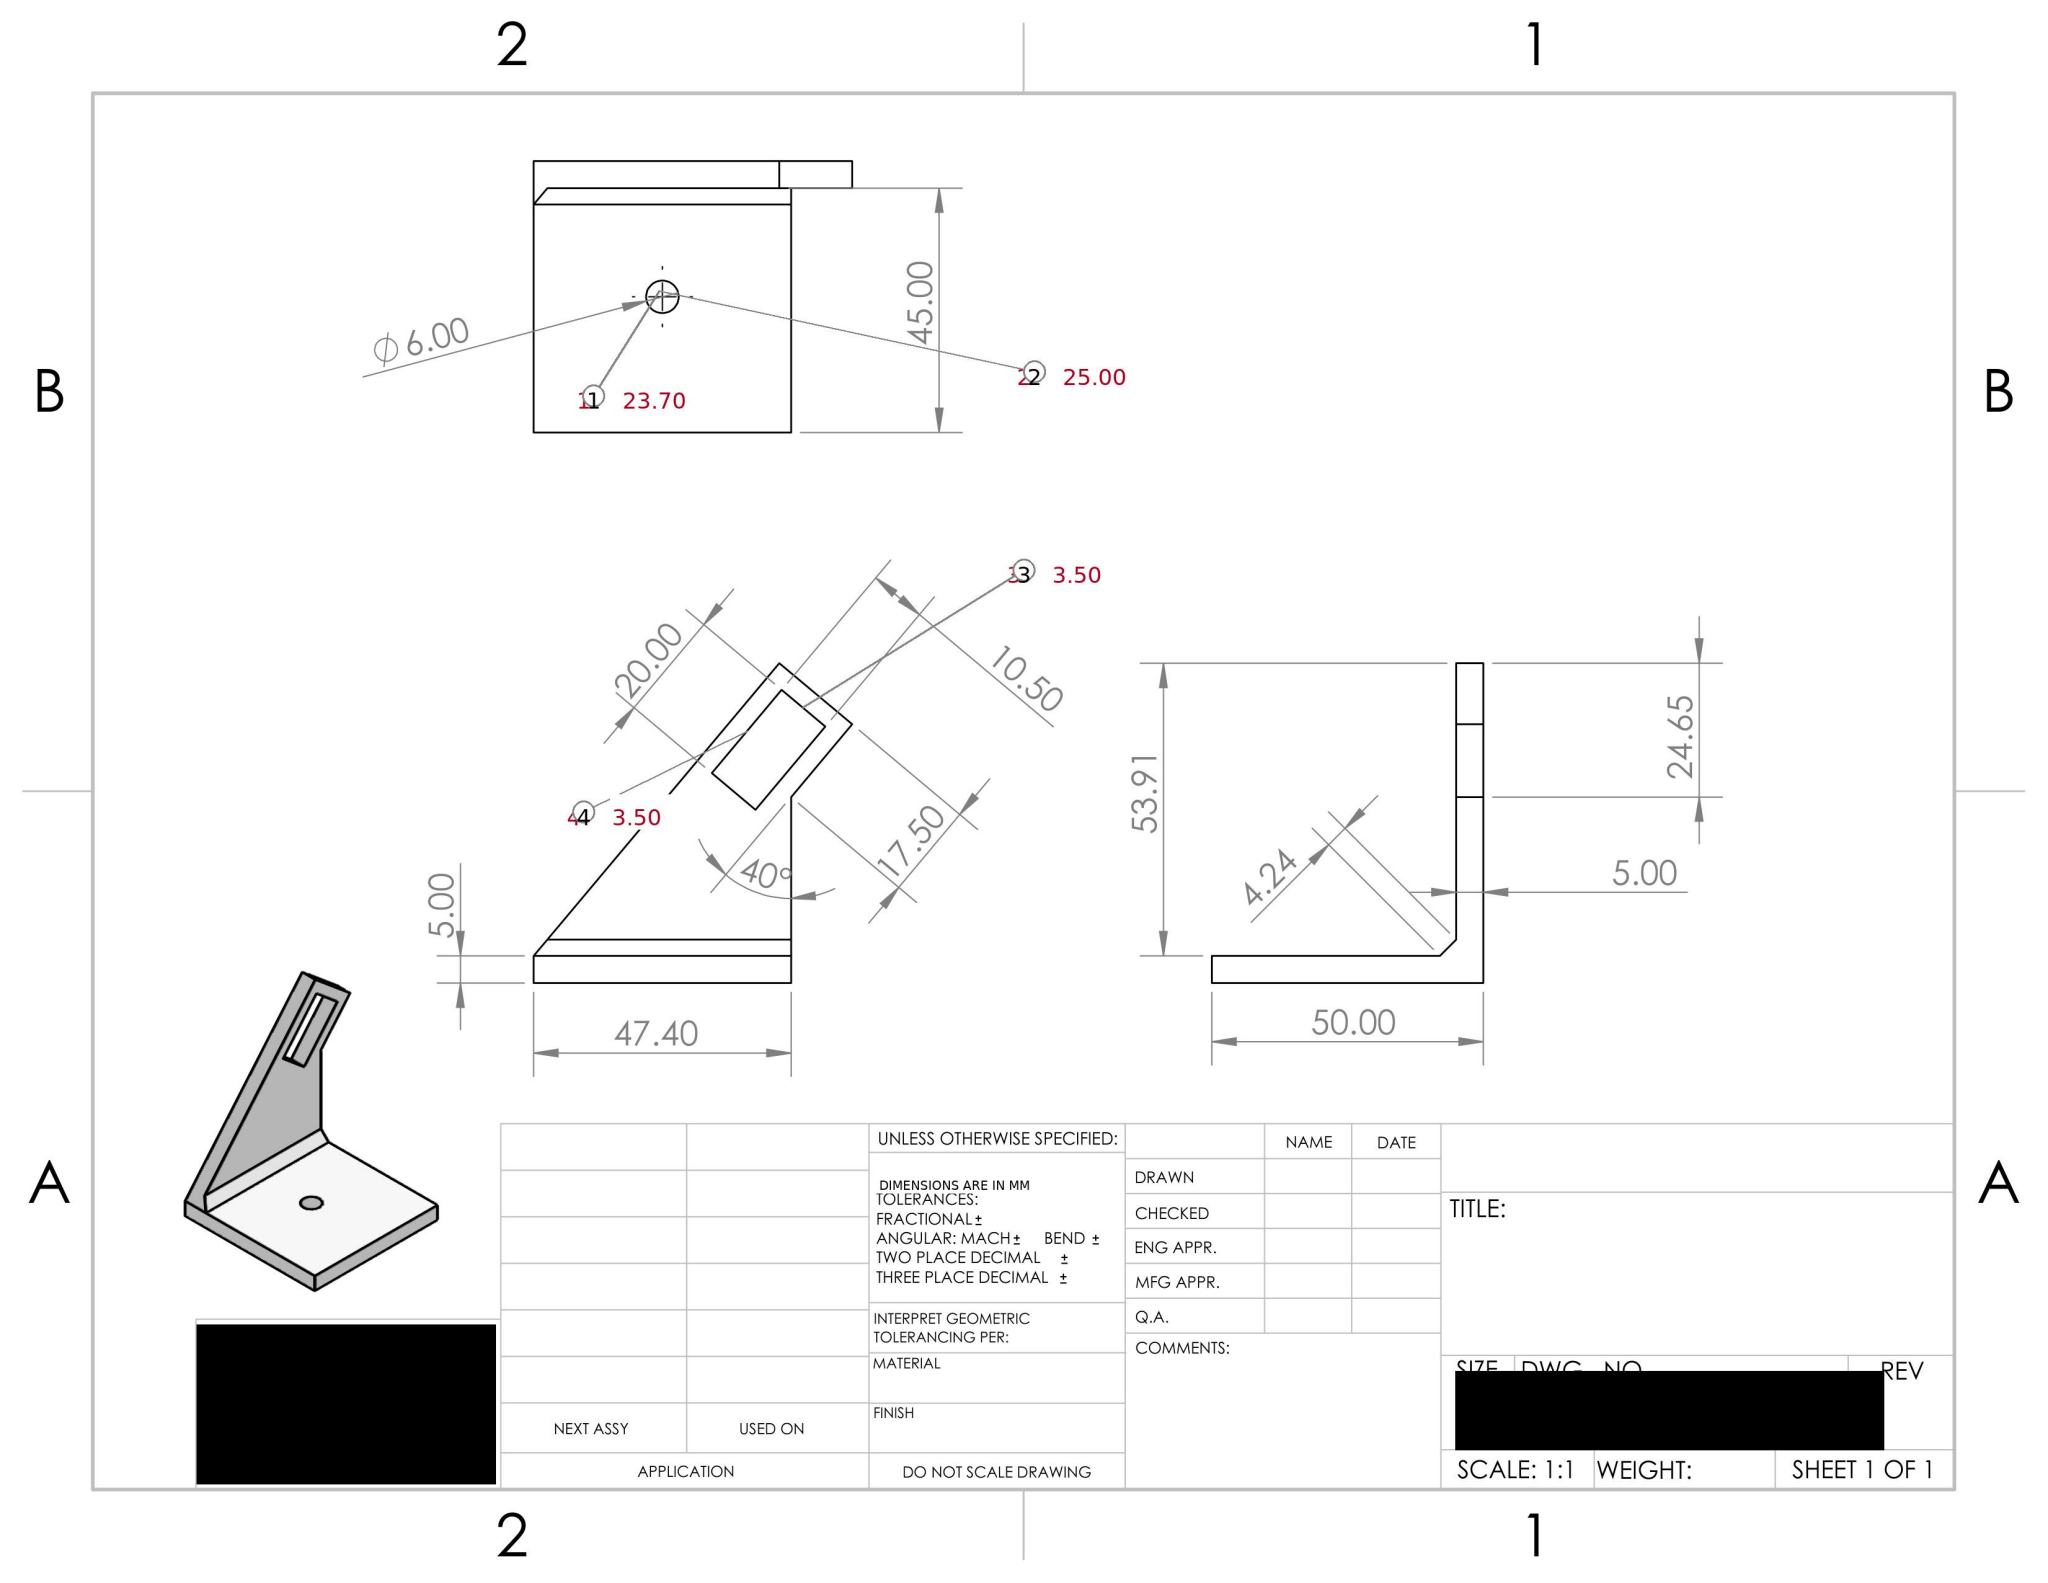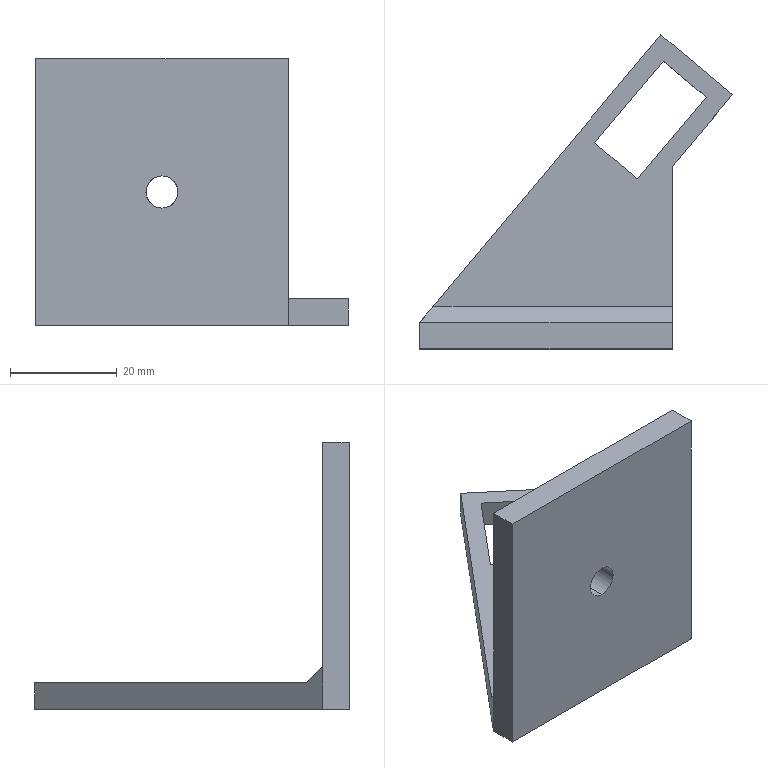Part | SolidWorks | mm | 1 solid | 17 faces | box 58.65 x 58.91 x 50 mm | volume 18179 mm3 | plane 15 | cylinder 2 | commonest cylinder face diameters 6 x2
STEP:
#1=CARTESIAN_POINT('',(23.698,0.,19.5));
#2=VERTEX_POINT('',#1);
#3=CARTESIAN_POINT('',(23.698,0.,25.5));
#4=VERTEX_POINT('',#3);
#5=CARTESIAN_POINT('',(23.698,0.,22.5));
#6=DIRECTION('',(0.,1.,0.));
#7=DIRECTION('',(0.,0.,1.));
#8=AXIS2_PLACEMENT_3D('',#5,#6,#7);
#9=CIRCLE('',#8,3.);
#10=EDGE_CURVE('',#2,#4,#9,.T.);
#11=ORIENTED_EDGE('',*,*,#10,.T.);
#12=CARTESIAN_POINT('',(23.698,-5.,25.5));
#13=VERTEX_POINT('',#12);
#14=CARTESIAN_POINT('',(23.698,53.914,25.5));
#15=DIRECTION('',(0.,-1.,0.));
#16=VECTOR('',#15,1000.);
#17=LINE('',#14,#16);
#18=EDGE_CURVE('',#4,#13,#17,.T.);
#19=ORIENTED_EDGE('',*,*,#18,.T.);
#20=CARTESIAN_POINT('',(23.698,-5.,19.5));
#21=VERTEX_POINT('',#20);
#22=CARTESIAN_POINT('',(23.698,-5.,25.5));
#23=CARTESIAN_POINT('',(23.305,-5.,25.5));
#24=CARTESIAN_POINT('',(22.913,-5.,25.422));
#25=CARTESIAN_POINT('',(22.187,-5.,25.121));
#26=CARTESIAN_POINT('',(21.854,-5.,24.899));
#27=CARTESIAN_POINT('',(21.299,-5.,24.344));
#28=CARTESIAN_POINT('',(21.077,-5.,24.011));
#29=CARTESIAN_POINT('',(20.776,-5.,23.285));
#30=CARTESIAN_POINT('',(20.698,-5.,22.893));
#31=CARTESIAN_POINT('',(20.698,-5.,22.107));
#32=CARTESIAN_POINT('',(20.776,-5.,21.715));
#33=CARTESIAN_POINT('',(21.077,-5.,20.989));
#34=CARTESIAN_POINT('',(21.299,-5.,20.656));
#35=CARTESIAN_POINT('',(21.854,-5.,20.101));
#36=CARTESIAN_POINT('',(22.187,-5.,19.879));
#37=CARTESIAN_POINT('',(22.913,-5.,19.578));
#38=CARTESIAN_POINT('',(23.305,-5.,19.5));
#39=CARTESIAN_POINT('',(23.698,-5.,19.5));
#40=B_SPLINE_CURVE_WITH_KNOTS('',3,(#22,#23,#24,#25,#26,#27,#28,#29,#30,#31,#32,#33,#34,#35,#36,#37,#38,#39),.UNSPECIFIED.,.F.,.F.,(4,2,2,2,2,2,2,2,4),(0.5,0.5625,0.625,0.6875,0.75,0.8125,0.875,0.9375,1.),.UNSPECIFIED.);
#41=EDGE_CURVE('',#13,#21,#40,.T.);
#42=ORIENTED_EDGE('',*,*,#41,.T.);
#43=CARTESIAN_POINT('',(23.698,53.914,19.5));
#44=DIRECTION('',(0.,-1.,0.));
#45=VECTOR('',#44,1000.);
#46=LINE('',#43,#45);
#47=EDGE_CURVE('',#2,#21,#46,.T.);
#48=ORIENTED_EDGE('',*,*,#47,.F.);
#49=EDGE_LOOP('',(#11,#19,#42,#48));
#50=FACE_OUTER_BOUND('',#49,.T.);
#51=CARTESIAN_POINT('',(23.698,53.914,22.5));
#52=DIRECTION('',(0.,-1.,0.));
#53=DIRECTION('',(0.,0.,-1.));
#54=AXIS2_PLACEMENT_3D('',#51,#52,#53);
#55=CYLINDRICAL_SURFACE('',#54,3.);
#56=ADVANCED_FACE('',(#50),#55,.F.);
#57=CARTESIAN_POINT('',(0.,-5.,47.5));
#58=VERTEX_POINT('',#57);
#59=CARTESIAN_POINT('',(0.,-5.,-2.5));
#60=VERTEX_POINT('',#59);
#61=CARTESIAN_POINT('',(0.,-5.,-2.5));
#62=DIRECTION('',(0.,0.,-1.));
#63=VECTOR('',#62,1000.);
#64=LINE('',#61,#63);
#65=EDGE_CURVE('',#58,#60,#64,.T.);
#66=ORIENTED_EDGE('',*,*,#65,.T.);
#67=CARTESIAN_POINT('',(47.396,-5.,-2.5));
#68=VERTEX_POINT('',#67);
#69=CARTESIAN_POINT('',(0.,-5.,-2.5));
#70=DIRECTION('',(1.,0.,0.));
#71=VECTOR('',#70,1000.);
#72=LINE('',#69,#71);
#73=EDGE_CURVE('',#60,#68,#72,.T.);
#74=ORIENTED_EDGE('',*,*,#73,.T.);
#75=CARTESIAN_POINT('',(47.396,-5.,47.5));
#76=VERTEX_POINT('',#75);
#77=CARTESIAN_POINT('',(47.396,-5.,-2.5));
#78=DIRECTION('',(0.,0.,1.));
#79=VECTOR('',#78,1000.);
#80=LINE('',#77,#79);
#81=EDGE_CURVE('',#68,#76,#80,.T.);
#82=ORIENTED_EDGE('',*,*,#81,.T.);
#83=CARTESIAN_POINT('',(0.,-5.,47.5));
#84=DIRECTION('',(-1.,0.,0.));
#85=VECTOR('',#84,1000.);
#86=LINE('',#83,#85);
#87=EDGE_CURVE('',#76,#58,#86,.T.);
#88=ORIENTED_EDGE('',*,*,#87,.T.);
#89=EDGE_LOOP('',(#66,#74,#82,#88));
#90=FACE_OUTER_BOUND('',#89,.T.);
#91=CARTESIAN_POINT('',(23.698,-5.,19.5));
#92=CARTESIAN_POINT('',(24.091,-5.,19.5));
#93=CARTESIAN_POINT('',(24.483,-5.,19.578));
#94=CARTESIAN_POINT('',(25.209,-5.,19.879));
#95=CARTESIAN_POINT('',(25.542,-5.,20.101));
#96=CARTESIAN_POINT('',(26.097,-5.,20.656));
#97=CARTESIAN_POINT('',(26.319,-5.,20.989));
#98=CARTESIAN_POINT('',(26.62,-5.,21.715));
#99=CARTESIAN_POINT('',(26.698,-5.,22.107));
#100=CARTESIAN_POINT('',(26.698,-5.,22.893));
#101=CARTESIAN_POINT('',(26.62,-5.,23.285));
#102=CARTESIAN_POINT('',(26.319,-5.,24.011));
#103=CARTESIAN_POINT('',(26.097,-5.,24.344));
#104=CARTESIAN_POINT('',(25.542,-5.,24.899));
#105=CARTESIAN_POINT('',(25.209,-5.,25.121));
#106=CARTESIAN_POINT('',(24.483,-5.,25.422));
#107=CARTESIAN_POINT('',(24.091,-5.,25.5));
#108=CARTESIAN_POINT('',(23.698,-5.,25.5));
#109=B_SPLINE_CURVE_WITH_KNOTS('',3,(#91,#92,#93,#94,#95,#96,#97,#98,#99,#100,#101,#102,#103,#104,#105,#106,#107,#108),.UNSPECIFIED.,.F.,.F.,(4,2,2,2,2,2,2,2,4),(0.,0.0625,0.125,0.1875,0.25,0.3125,0.375,0.4375,0.5),.UNSPECIFIED.);
#110=EDGE_CURVE('',#21,#13,#109,.T.);
#111=ORIENTED_EDGE('',*,*,#110,.F.);
#112=ORIENTED_EDGE('',*,*,#41,.F.);
#113=EDGE_LOOP('',(#111,#112));
#114=FACE_BOUND('',#113,.T.);
#115=CARTESIAN_POINT('',(0.,-5.,0.));
#116=DIRECTION('',(0.,1.,0.));
#117=DIRECTION('',(0.,0.,1.));
#118=AXIS2_PLACEMENT_3D('',#115,#116,#117);
#119=PLANE('',#118);
#120=ADVANCED_FACE('',(#90,#114),#119,.F.);
#121=CARTESIAN_POINT('',(45.239,53.914,2.5));
#122=VERTEX_POINT('',#121);
#123=CARTESIAN_POINT('',(2.517,3.,2.5));
#124=VERTEX_POINT('',#123);
#125=CARTESIAN_POINT('',(0.,0.,2.5));
#126=DIRECTION('',(-0.6428,-0.766,0.));
#127=VECTOR('',#126,1000.);
#128=LINE('',#125,#127);
#129=EDGE_CURVE('',#122,#124,#128,.T.);
#130=ORIENTED_EDGE('',*,*,#129,.T.);
#131=CARTESIAN_POINT('',(47.396,3.,2.5));
#132=VERTEX_POINT('',#131);
#133=CARTESIAN_POINT('',(0.,3.,2.5));
#134=DIRECTION('',(1.,0.,0.));
#135=VECTOR('',#134,1000.);
#136=LINE('',#133,#135);
#137=EDGE_CURVE('',#124,#132,#136,.T.);
#138=ORIENTED_EDGE('',*,*,#137,.T.);
#139=CARTESIAN_POINT('',(47.396,29.259,2.5));
#140=VERTEX_POINT('',#139);
#141=CARTESIAN_POINT('',(47.396,29.259,2.5));
#142=DIRECTION('',(0.,1.,0.));
#143=VECTOR('',#142,1000.);
#144=LINE('',#141,#143);
#145=EDGE_CURVE('',#132,#140,#144,.T.);
#146=ORIENTED_EDGE('',*,*,#145,.T.);
#147=CARTESIAN_POINT('',(58.645,42.665,2.5));
#148=VERTEX_POINT('',#147);
#149=CARTESIAN_POINT('',(58.645,42.665,2.5));
#150=DIRECTION('',(0.6428,0.766,0.));
#151=VECTOR('',#150,1000.);
#152=LINE('',#149,#151);
#153=EDGE_CURVE('',#140,#148,#152,.T.);
#154=ORIENTED_EDGE('',*,*,#153,.T.);
#155=CARTESIAN_POINT('',(45.239,53.914,2.5));
#156=DIRECTION('',(-0.766,0.6428,0.));
#157=VECTOR('',#156,1000.);
#158=LINE('',#155,#157);
#159=EDGE_CURVE('',#148,#122,#158,.T.);
#160=ORIENTED_EDGE('',*,*,#159,.T.);
#161=EDGE_LOOP('',(#130,#138,#146,#154,#160));
#162=FACE_OUTER_BOUND('',#161,.T.);
#163=CARTESIAN_POINT('',(53.714,42.234,2.5));
#164=VERTEX_POINT('',#163);
#165=CARTESIAN_POINT('',(45.671,48.983,2.5));
#166=VERTEX_POINT('',#165);
#167=CARTESIAN_POINT('',(45.671,48.983,2.5));
#168=DIRECTION('',(-0.766,0.6428,0.));
#169=VECTOR('',#168,1000.);
#170=LINE('',#167,#169);
#171=EDGE_CURVE('',#164,#166,#170,.T.);
#172=ORIENTED_EDGE('',*,*,#171,.F.);
#173=CARTESIAN_POINT('',(40.858,26.913,2.5));
#174=VERTEX_POINT('',#173);
#175=CARTESIAN_POINT('',(53.714,42.234,2.5));
#176=DIRECTION('',(0.6428,0.766,0.));
#177=VECTOR('',#176,1000.);
#178=LINE('',#175,#177);
#179=EDGE_CURVE('',#174,#164,#178,.T.);
#180=ORIENTED_EDGE('',*,*,#179,.F.);
#181=CARTESIAN_POINT('',(32.815,33.662,2.5));
#182=VERTEX_POINT('',#181);
#183=CARTESIAN_POINT('',(32.815,33.662,2.5));
#184=DIRECTION('',(0.766,-0.6428,0.));
#185=VECTOR('',#184,1000.);
#186=LINE('',#183,#185);
#187=EDGE_CURVE('',#182,#174,#186,.T.);
#188=ORIENTED_EDGE('',*,*,#187,.F.);
#189=CARTESIAN_POINT('',(45.671,48.983,2.5));
#190=DIRECTION('',(-0.6428,-0.766,0.));
#191=VECTOR('',#190,1000.);
#192=LINE('',#189,#191);
#193=EDGE_CURVE('',#166,#182,#192,.T.);
#194=ORIENTED_EDGE('',*,*,#193,.F.);
#195=EDGE_LOOP('',(#172,#180,#188,#194));
#196=FACE_BOUND('',#195,.T.);
#197=CARTESIAN_POINT('',(0.,0.,2.5));
#198=DIRECTION('',(0.,0.,-1.));
#199=DIRECTION('',(-1.,0.,0.));
#200=AXIS2_PLACEMENT_3D('',#197,#198,#199);
#201=PLANE('',#200);
#202=ADVANCED_FACE('',(#162,#196),#201,.F.);
#203=CARTESIAN_POINT('',(47.396,29.259,-2.5));
#204=VERTEX_POINT('',#203);
#205=CARTESIAN_POINT('',(47.396,29.259,-2.5));
#206=DIRECTION('',(0.,1.,0.));
#207=VECTOR('',#206,1000.);
#208=LINE('',#205,#207);
#209=EDGE_CURVE('',#68,#204,#208,.T.);
#210=ORIENTED_EDGE('',*,*,#209,.F.);
#211=ORIENTED_EDGE('',*,*,#73,.F.);
#212=CARTESIAN_POINT('',(0.,0.,-2.5));
#213=VERTEX_POINT('',#212);
#214=CARTESIAN_POINT('',(0.,-5.,-2.5));
#215=DIRECTION('',(0.,1.,0.));
#216=VECTOR('',#215,1000.);
#217=LINE('',#214,#216);
#218=EDGE_CURVE('',#60,#213,#217,.T.);
#219=ORIENTED_EDGE('',*,*,#218,.T.);
#220=CARTESIAN_POINT('',(45.239,53.914,-2.5));
#221=VERTEX_POINT('',#220);
#222=CARTESIAN_POINT('',(0.,0.,-2.5));
#223=DIRECTION('',(-0.6428,-0.766,0.));
#224=VECTOR('',#223,1000.);
#225=LINE('',#222,#224);
#226=EDGE_CURVE('',#221,#213,#225,.T.);
#227=ORIENTED_EDGE('',*,*,#226,.F.);
#228=CARTESIAN_POINT('',(58.645,42.665,-2.5));
#229=VERTEX_POINT('',#228);
#230=CARTESIAN_POINT('',(45.239,53.914,-2.5));
#231=DIRECTION('',(-0.766,0.6428,0.));
#232=VECTOR('',#231,1000.);
#233=LINE('',#230,#232);
#234=EDGE_CURVE('',#229,#221,#233,.T.);
#235=ORIENTED_EDGE('',*,*,#234,.F.);
#236=CARTESIAN_POINT('',(58.645,42.665,-2.5));
#237=DIRECTION('',(0.6428,0.766,0.));
#238=VECTOR('',#237,1000.);
#239=LINE('',#236,#238);
#240=EDGE_CURVE('',#204,#229,#239,.T.);
#241=ORIENTED_EDGE('',*,*,#240,.F.);
#242=EDGE_LOOP('',(#210,#211,#219,#227,#235,#241));
#243=FACE_OUTER_BOUND('',#242,.T.);
#244=CARTESIAN_POINT('',(40.858,26.913,-2.5));
#245=VERTEX_POINT('',#244);
#246=CARTESIAN_POINT('',(53.714,42.234,-2.5));
#247=VERTEX_POINT('',#246);
#248=CARTESIAN_POINT('',(53.714,42.234,-2.5));
#249=DIRECTION('',(0.6428,0.766,0.));
#250=VECTOR('',#249,1000.);
#251=LINE('',#248,#250);
#252=EDGE_CURVE('',#245,#247,#251,.T.);
#253=ORIENTED_EDGE('',*,*,#252,.T.);
#254=CARTESIAN_POINT('',(45.671,48.983,-2.5));
#255=VERTEX_POINT('',#254);
#256=CARTESIAN_POINT('',(45.671,48.983,-2.5));
#257=DIRECTION('',(-0.766,0.6428,0.));
#258=VECTOR('',#257,1000.);
#259=LINE('',#256,#258);
#260=EDGE_CURVE('',#247,#255,#259,.T.);
#261=ORIENTED_EDGE('',*,*,#260,.T.);
#262=CARTESIAN_POINT('',(32.815,33.662,-2.5));
#263=VERTEX_POINT('',#262);
#264=CARTESIAN_POINT('',(45.671,48.983,-2.5));
#265=DIRECTION('',(-0.6428,-0.766,0.));
#266=VECTOR('',#265,1000.);
#267=LINE('',#264,#266);
#268=EDGE_CURVE('',#255,#263,#267,.T.);
#269=ORIENTED_EDGE('',*,*,#268,.T.);
#270=CARTESIAN_POINT('',(32.815,33.662,-2.5));
#271=DIRECTION('',(0.766,-0.6428,0.));
#272=VECTOR('',#271,1000.);
#273=LINE('',#270,#272);
#274=EDGE_CURVE('',#263,#245,#273,.T.);
#275=ORIENTED_EDGE('',*,*,#274,.T.);
#276=EDGE_LOOP('',(#253,#261,#269,#275));
#277=FACE_BOUND('',#276,.T.);
#278=CARTESIAN_POINT('',(0.,0.,-2.5));
#279=DIRECTION('',(0.,0.,-1.));
#280=DIRECTION('',(-1.,0.,0.));
#281=AXIS2_PLACEMENT_3D('',#278,#279,#280);
#282=PLANE('',#281);
#283=ADVANCED_FACE('',(#243,#277),#282,.T.);
#284=ORIENTED_EDGE('',*,*,#209,.T.);
#285=CARTESIAN_POINT('',(47.396,29.259,2.5));
#286=DIRECTION('',(0.,0.,-1.));
#287=VECTOR('',#286,1000.);
#288=LINE('',#285,#287);
#289=EDGE_CURVE('',#140,#204,#288,.T.);
#290=ORIENTED_EDGE('',*,*,#289,.F.);
#291=ORIENTED_EDGE('',*,*,#145,.F.);
#292=CARTESIAN_POINT('',(47.396,0.,5.5));
#293=VERTEX_POINT('',#292);
#294=CARTESIAN_POINT('',(47.396,16.13,-10.63));
#295=DIRECTION('',(0.,-0.7071,0.7071));
#296=VECTOR('',#295,1000.);
#297=LINE('',#294,#296);
#298=EDGE_CURVE('',#132,#293,#297,.T.);
#299=ORIENTED_EDGE('',*,*,#298,.T.);
#300=CARTESIAN_POINT('',(47.396,0.,47.5));
#301=VERTEX_POINT('',#300);
#302=CARTESIAN_POINT('',(47.396,0.,-2.5));
#303=DIRECTION('',(0.,0.,1.));
#304=VECTOR('',#303,1000.);
#305=LINE('',#302,#304);
#306=EDGE_CURVE('',#293,#301,#305,.T.);
#307=ORIENTED_EDGE('',*,*,#306,.T.);
#308=CARTESIAN_POINT('',(47.396,-5.,47.5));
#309=DIRECTION('',(0.,1.,0.));
#310=VECTOR('',#309,1000.);
#311=LINE('',#308,#310);
#312=EDGE_CURVE('',#76,#301,#311,.T.);
#313=ORIENTED_EDGE('',*,*,#312,.F.);
#314=ORIENTED_EDGE('',*,*,#81,.F.);
#315=EDGE_LOOP('',(#284,#290,#291,#299,#307,#313,#314));
#316=FACE_OUTER_BOUND('',#315,.T.);
#317=CARTESIAN_POINT('',(47.396,29.259,2.5));
#318=DIRECTION('',(-1.,0.,0.));
#319=DIRECTION('',(0.,0.,1.));
#320=AXIS2_PLACEMENT_3D('',#317,#318,#319);
#321=PLANE('',#320);
#322=ADVANCED_FACE('',(#316),#321,.F.);
#323=ORIENTED_EDGE('',*,*,#240,.T.);
#324=CARTESIAN_POINT('',(58.645,42.665,2.5));
#325=DIRECTION('',(0.,0.,-1.));
#326=VECTOR('',#325,1000.);
#327=LINE('',#324,#326);
#328=EDGE_CURVE('',#148,#229,#327,.T.);
#329=ORIENTED_EDGE('',*,*,#328,.F.);
#330=ORIENTED_EDGE('',*,*,#153,.F.);
#331=ORIENTED_EDGE('',*,*,#289,.T.);
#332=EDGE_LOOP('',(#323,#329,#330,#331));
#333=FACE_OUTER_BOUND('',#332,.T.);
#334=CARTESIAN_POINT('',(58.645,42.665,2.5));
#335=DIRECTION('',(-0.766,0.6428,0.));
#336=DIRECTION('',(-0.6428,-0.766,0.));
#337=AXIS2_PLACEMENT_3D('',#334,#335,#336);
#338=PLANE('',#337);
#339=ADVANCED_FACE('',(#333),#338,.F.);
#340=ORIENTED_EDGE('',*,*,#234,.T.);
#341=CARTESIAN_POINT('',(45.239,53.914,2.5));
#342=DIRECTION('',(0.,0.,-1.));
#343=VECTOR('',#342,1000.);
#344=LINE('',#341,#343);
#345=EDGE_CURVE('',#122,#221,#344,.T.);
#346=ORIENTED_EDGE('',*,*,#345,.F.);
#347=ORIENTED_EDGE('',*,*,#159,.F.);
#348=ORIENTED_EDGE('',*,*,#328,.T.);
#349=EDGE_LOOP('',(#340,#346,#347,#348));
#350=FACE_OUTER_BOUND('',#349,.T.);
#351=CARTESIAN_POINT('',(45.239,53.914,2.5));
#352=DIRECTION('',(-0.6428,-0.766,0.));
#353=DIRECTION('',(0.766,-0.6428,0.));
#354=AXIS2_PLACEMENT_3D('',#351,#352,#353);
#355=PLANE('',#354);
#356=ADVANCED_FACE('',(#350),#355,.F.);
#357=ORIENTED_EDGE('',*,*,#226,.T.);
#358=CARTESIAN_POINT('',(0.,0.,5.5));
#359=VERTEX_POINT('',#358);
#360=CARTESIAN_POINT('',(0.,0.,2.5));
#361=DIRECTION('',(0.,0.,-1.));
#362=VECTOR('',#361,1000.);
#363=LINE('',#360,#362);
#364=EDGE_CURVE('',#359,#213,#363,.T.);
#365=ORIENTED_EDGE('',*,*,#364,.F.);
#366=CARTESIAN_POINT('',(0.9309,1.109,4.391));
#367=DIRECTION('',(0.5103,0.6081,-0.6081));
#368=VECTOR('',#367,1000.);
#369=LINE('',#366,#368);
#370=EDGE_CURVE('',#359,#124,#369,.T.);
#371=ORIENTED_EDGE('',*,*,#370,.T.);
#372=ORIENTED_EDGE('',*,*,#129,.F.);
#373=ORIENTED_EDGE('',*,*,#345,.T.);
#374=EDGE_LOOP('',(#357,#365,#371,#372,#373));
#375=FACE_OUTER_BOUND('',#374,.T.);
#376=CARTESIAN_POINT('',(0.,0.,2.5));
#377=DIRECTION('',(0.766,-0.6428,0.));
#378=DIRECTION('',(0.6428,0.766,0.));
#379=AXIS2_PLACEMENT_3D('',#376,#377,#378);
#380=PLANE('',#379);
#381=ADVANCED_FACE('',(#375),#380,.F.);
#382=ORIENTED_EDGE('',*,*,#260,.F.);
#383=CARTESIAN_POINT('',(53.714,42.234,2.5));
#384=DIRECTION('',(0.,0.,-1.));
#385=VECTOR('',#384,1000.);
#386=LINE('',#383,#385);
#387=EDGE_CURVE('',#164,#247,#386,.T.);
#388=ORIENTED_EDGE('',*,*,#387,.F.);
#389=ORIENTED_EDGE('',*,*,#171,.T.);
#390=CARTESIAN_POINT('',(45.671,48.983,2.5));
#391=DIRECTION('',(0.,0.,-1.));
#392=VECTOR('',#391,1000.);
#393=LINE('',#390,#392);
#394=EDGE_CURVE('',#166,#255,#393,.T.);
#395=ORIENTED_EDGE('',*,*,#394,.T.);
#396=EDGE_LOOP('',(#382,#388,#389,#395));
#397=FACE_OUTER_BOUND('',#396,.T.);
#398=CARTESIAN_POINT('',(45.671,48.983,2.5));
#399=DIRECTION('',(-0.6428,-0.766,0.));
#400=DIRECTION('',(0.766,-0.6428,0.));
#401=AXIS2_PLACEMENT_3D('',#398,#399,#400);
#402=PLANE('',#401);
#403=ADVANCED_FACE('',(#397),#402,.T.);
#404=ORIENTED_EDGE('',*,*,#268,.F.);
#405=ORIENTED_EDGE('',*,*,#394,.F.);
#406=ORIENTED_EDGE('',*,*,#193,.T.);
#407=CARTESIAN_POINT('',(32.815,33.662,2.5));
#408=DIRECTION('',(0.,0.,-1.));
#409=VECTOR('',#408,1000.);
#410=LINE('',#407,#409);
#411=EDGE_CURVE('',#182,#263,#410,.T.);
#412=ORIENTED_EDGE('',*,*,#411,.T.);
#413=EDGE_LOOP('',(#404,#405,#406,#412));
#414=FACE_OUTER_BOUND('',#413,.T.);
#415=CARTESIAN_POINT('',(45.671,48.983,2.5));
#416=DIRECTION('',(0.766,-0.6428,0.));
#417=DIRECTION('',(0.6428,0.766,0.));
#418=AXIS2_PLACEMENT_3D('',#415,#416,#417);
#419=PLANE('',#418);
#420=ADVANCED_FACE('',(#414),#419,.T.);
#421=ORIENTED_EDGE('',*,*,#274,.F.);
#422=ORIENTED_EDGE('',*,*,#411,.F.);
#423=ORIENTED_EDGE('',*,*,#187,.T.);
#424=CARTESIAN_POINT('',(40.858,26.913,2.5));
#425=DIRECTION('',(0.,0.,-1.));
#426=VECTOR('',#425,1000.);
#427=LINE('',#424,#426);
#428=EDGE_CURVE('',#174,#245,#427,.T.);
#429=ORIENTED_EDGE('',*,*,#428,.T.);
#430=EDGE_LOOP('',(#421,#422,#423,#429));
#431=FACE_OUTER_BOUND('',#430,.T.);
#432=CARTESIAN_POINT('',(32.815,33.662,2.5));
#433=DIRECTION('',(0.6428,0.766,0.));
#434=DIRECTION('',(-0.766,0.6428,0.));
#435=AXIS2_PLACEMENT_3D('',#432,#433,#434);
#436=PLANE('',#435);
#437=ADVANCED_FACE('',(#431),#436,.T.);
#438=ORIENTED_EDGE('',*,*,#252,.F.);
#439=ORIENTED_EDGE('',*,*,#428,.F.);
#440=ORIENTED_EDGE('',*,*,#179,.T.);
#441=ORIENTED_EDGE('',*,*,#387,.T.);
#442=EDGE_LOOP('',(#438,#439,#440,#441));
#443=FACE_OUTER_BOUND('',#442,.T.);
#444=CARTESIAN_POINT('',(53.714,42.234,2.5));
#445=DIRECTION('',(-0.766,0.6428,0.));
#446=DIRECTION('',(-0.6428,-0.766,0.));
#447=AXIS2_PLACEMENT_3D('',#444,#445,#446);
#448=PLANE('',#447);
#449=ADVANCED_FACE('',(#443),#448,.T.);
#450=ORIENTED_EDGE('',*,*,#10,.F.);
#451=CARTESIAN_POINT('',(23.698,0.,22.5));
#452=DIRECTION('',(0.,1.,0.));
#453=DIRECTION('',(0.,0.,1.));
#454=AXIS2_PLACEMENT_3D('',#451,#452,#453);
#455=CIRCLE('',#454,3.);
#456=EDGE_CURVE('',#4,#2,#455,.T.);
#457=ORIENTED_EDGE('',*,*,#456,.F.);
#458=EDGE_LOOP('',(#450,#457));
#459=FACE_BOUND('',#458,.T.);
#460=ORIENTED_EDGE('',*,*,#306,.F.);
#461=CARTESIAN_POINT('',(0.,0.,5.5));
#462=DIRECTION('',(-1.,0.,0.));
#463=VECTOR('',#462,1000.);
#464=LINE('',#461,#463);
#465=EDGE_CURVE('',#293,#359,#464,.T.);
#466=ORIENTED_EDGE('',*,*,#465,.T.);
#467=CARTESIAN_POINT('',(0.,0.,47.5));
#468=VERTEX_POINT('',#467);
#469=CARTESIAN_POINT('',(0.,0.,-2.5));
#470=DIRECTION('',(0.,0.,-1.));
#471=VECTOR('',#470,1000.);
#472=LINE('',#469,#471);
#473=EDGE_CURVE('',#468,#359,#472,.T.);
#474=ORIENTED_EDGE('',*,*,#473,.F.);
#475=CARTESIAN_POINT('',(0.,0.,47.5));
#476=DIRECTION('',(-1.,0.,0.));
#477=VECTOR('',#476,1000.);
#478=LINE('',#475,#477);
#479=EDGE_CURVE('',#301,#468,#478,.T.);
#480=ORIENTED_EDGE('',*,*,#479,.F.);
#481=EDGE_LOOP('',(#460,#466,#474,#480));
#482=FACE_OUTER_BOUND('',#481,.T.);
#483=CARTESIAN_POINT('',(0.,0.,0.));
#484=DIRECTION('',(0.,1.,0.));
#485=DIRECTION('',(0.,0.,1.));
#486=AXIS2_PLACEMENT_3D('',#483,#484,#485);
#487=PLANE('',#486);
#488=ADVANCED_FACE('',(#459,#482),#487,.T.);
#489=ORIENTED_EDGE('',*,*,#473,.T.);
#490=ORIENTED_EDGE('',*,*,#364,.T.);
#491=ORIENTED_EDGE('',*,*,#218,.F.);
#492=ORIENTED_EDGE('',*,*,#65,.F.);
#493=CARTESIAN_POINT('',(0.,-5.,47.5));
#494=DIRECTION('',(0.,1.,0.));
#495=VECTOR('',#494,1000.);
#496=LINE('',#493,#495);
#497=EDGE_CURVE('',#58,#468,#496,.T.);
#498=ORIENTED_EDGE('',*,*,#497,.T.);
#499=EDGE_LOOP('',(#489,#490,#491,#492,#498));
#500=FACE_OUTER_BOUND('',#499,.T.);
#501=CARTESIAN_POINT('',(0.,-5.,-2.5));
#502=DIRECTION('',(1.,0.,0.));
#503=DIRECTION('',(0.,0.,-1.));
#504=AXIS2_PLACEMENT_3D('',#501,#502,#503);
#505=PLANE('',#504);
#506=ADVANCED_FACE('',(#500),#505,.F.);
#507=ORIENTED_EDGE('',*,*,#479,.T.);
#508=ORIENTED_EDGE('',*,*,#497,.F.);
#509=ORIENTED_EDGE('',*,*,#87,.F.);
#510=ORIENTED_EDGE('',*,*,#312,.T.);
#511=EDGE_LOOP('',(#507,#508,#509,#510));
#512=FACE_OUTER_BOUND('',#511,.T.);
#513=CARTESIAN_POINT('',(0.,-5.,47.5));
#514=DIRECTION('',(0.,0.,-1.));
#515=DIRECTION('',(-1.,0.,0.));
#516=AXIS2_PLACEMENT_3D('',#513,#514,#515);
#517=PLANE('',#516);
#518=ADVANCED_FACE('',(#512),#517,.F.);
#519=ORIENTED_EDGE('',*,*,#370,.F.);
#520=ORIENTED_EDGE('',*,*,#465,.F.);
#521=ORIENTED_EDGE('',*,*,#298,.F.);
#522=ORIENTED_EDGE('',*,*,#137,.F.);
#523=EDGE_LOOP('',(#519,#520,#521,#522));
#524=FACE_OUTER_BOUND('',#523,.T.);
#525=CARTESIAN_POINT('',(0.,3.,2.5));
#526=DIRECTION('',(0.,-0.7071,-0.7071));
#527=DIRECTION('',(1.,0.,0.));
#528=AXIS2_PLACEMENT_3D('',#525,#526,#527);
#529=PLANE('',#528);
#530=ADVANCED_FACE('',(#524),#529,.F.);
#531=ORIENTED_EDGE('',*,*,#18,.F.);
#532=ORIENTED_EDGE('',*,*,#456,.T.);
#533=ORIENTED_EDGE('',*,*,#47,.T.);
#534=ORIENTED_EDGE('',*,*,#110,.T.);
#535=EDGE_LOOP('',(#531,#532,#533,#534));
#536=FACE_OUTER_BOUND('',#535,.T.);
#537=CARTESIAN_POINT('',(23.698,53.914,22.5));
#538=DIRECTION('',(0.,-1.,0.));
#539=DIRECTION('',(0.,0.,-1.));
#540=AXIS2_PLACEMENT_3D('',#537,#538,#539);
#541=CYLINDRICAL_SURFACE('',#540,3.);
#542=ADVANCED_FACE('',(#536),#541,.F.);
#543=CLOSED_SHELL('',(#56,#120,#202,#283,#322,#339,#356,#381,#403,#420,#437,#449,#488,#506,#518,#530,#542));
#544=MANIFOLD_SOLID_BREP('',#543);
#545=CARTESIAN_POINT('',(0.,0.,0.));
#546=DIRECTION('',(0.,0.,1.));
#547=DIRECTION('',(1.,0.,0.));
#548=AXIS2_PLACEMENT_3D('',#545,#546,#547);
#549=(LENGTH_UNIT()NAMED_UNIT(*)SI_UNIT(.MILLI.,.METRE.));
#550=UNCERTAINTY_MEASURE_WITH_UNIT(LENGTH_MEASURE(0.00001),#549,'','');
#551=(NAMED_UNIT(*)PLANE_ANGLE_UNIT()SI_UNIT($,.RADIAN.));
#552=(NAMED_UNIT(*)SI_UNIT($,.STERADIAN.)SOLID_ANGLE_UNIT());
#553=(GEOMETRIC_REPRESENTATION_CONTEXT(3)GLOBAL_UNCERTAINTY_ASSIGNED_CONTEXT((#550))GLOBAL_UNIT_ASSIGNED_CONTEXT((#549,#551,#552))REPRESENTATION_CONTEXT('',''));
#554=ADVANCED_BREP_SHAPE_REPRESENTATION('',(#544,#548),#553);